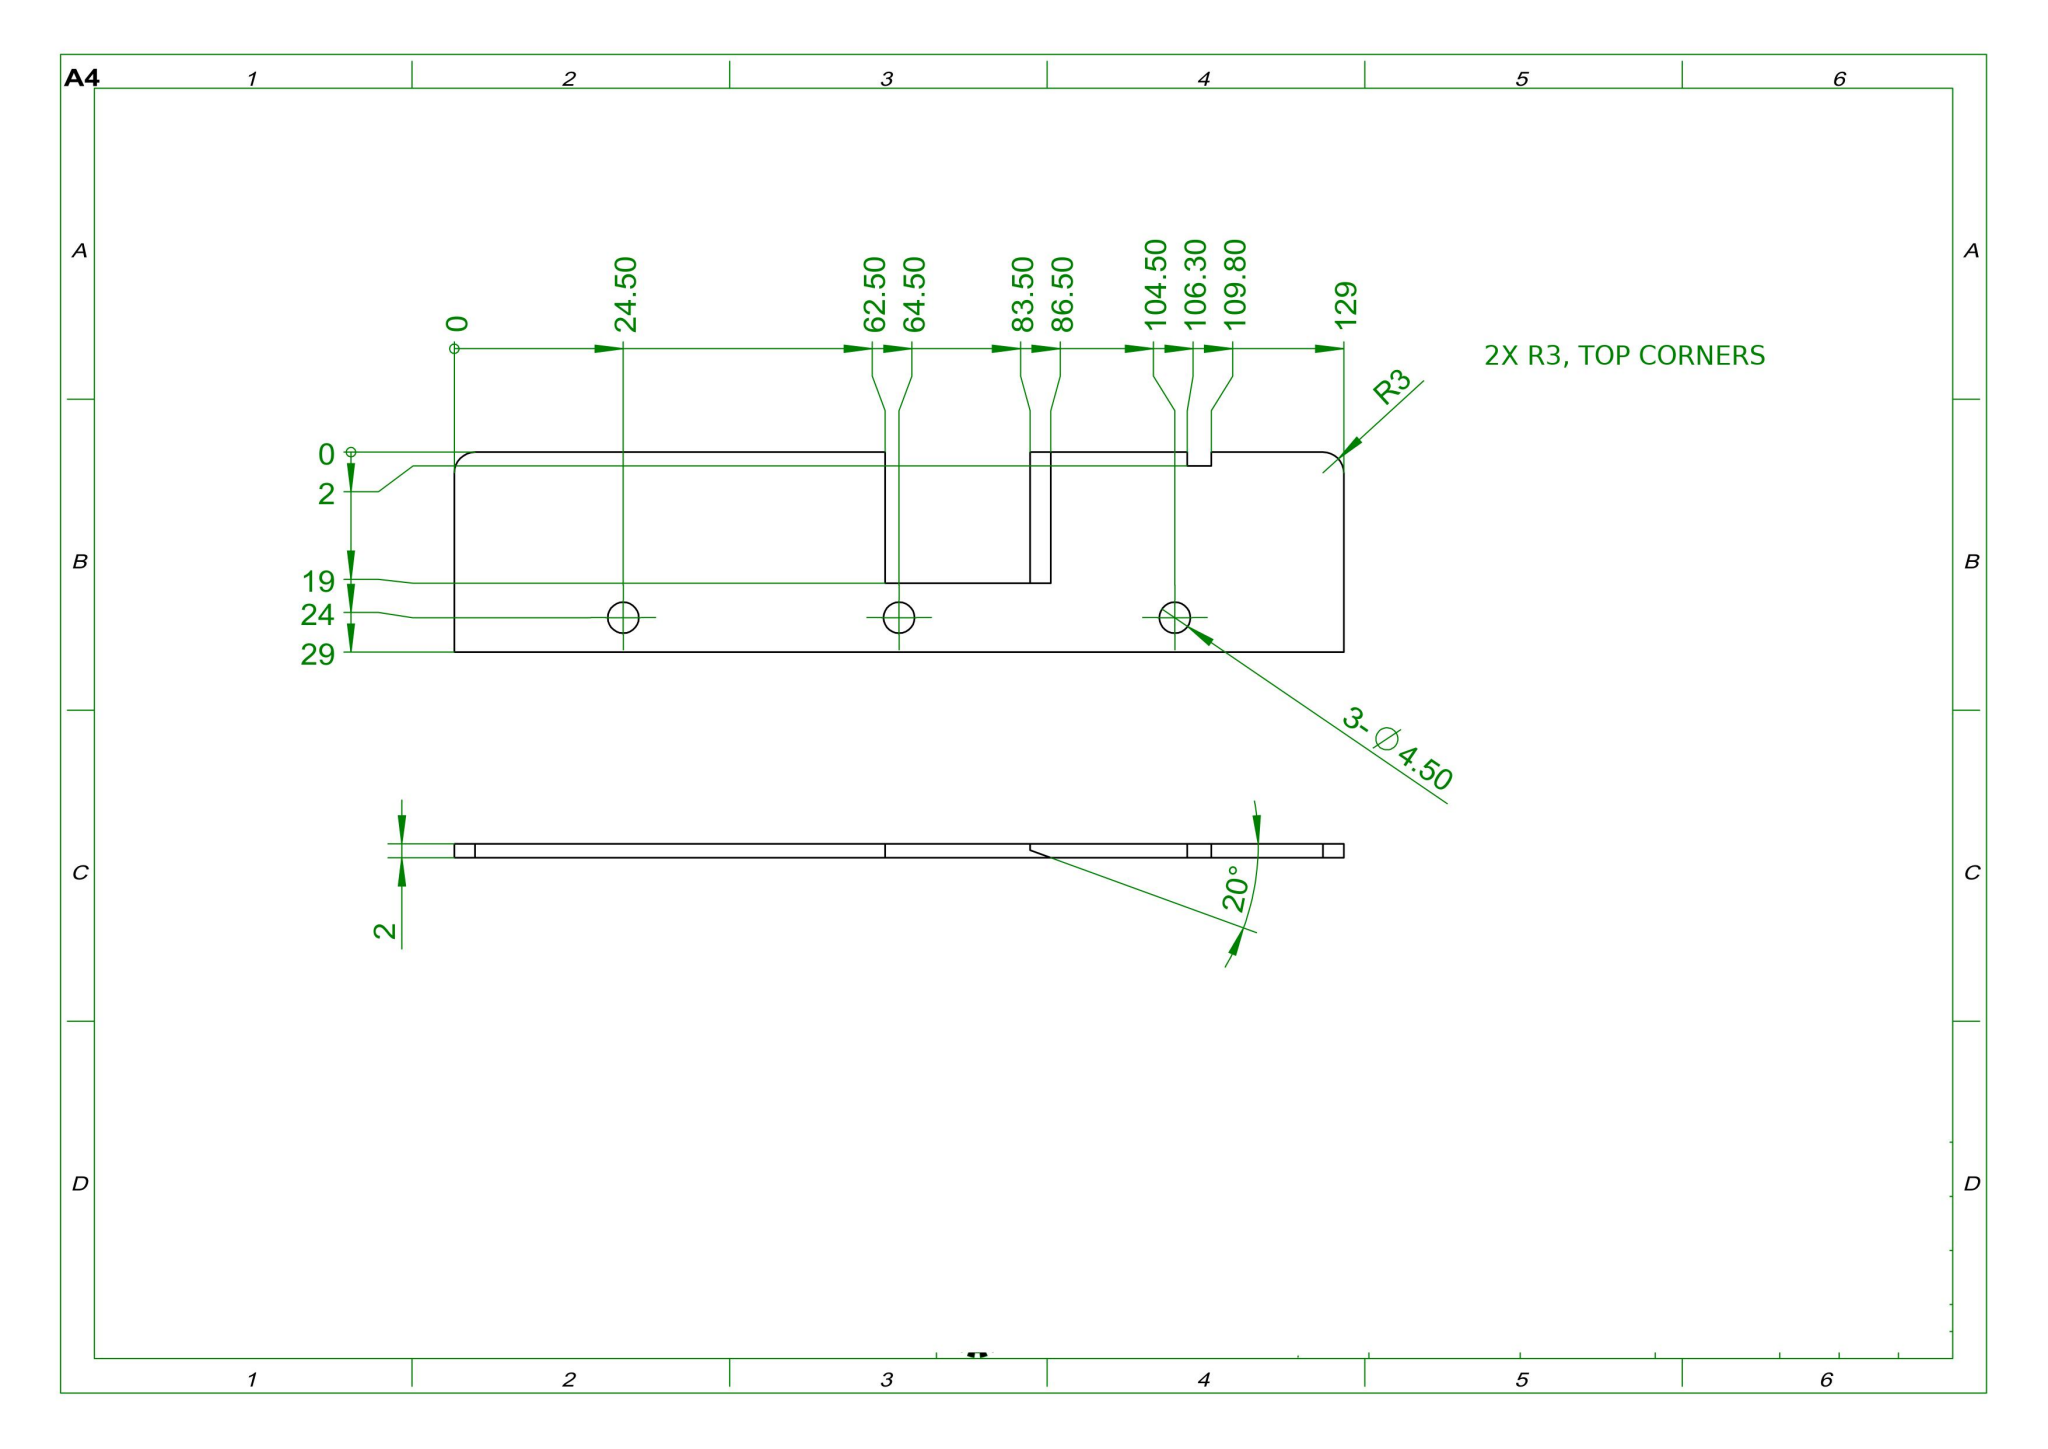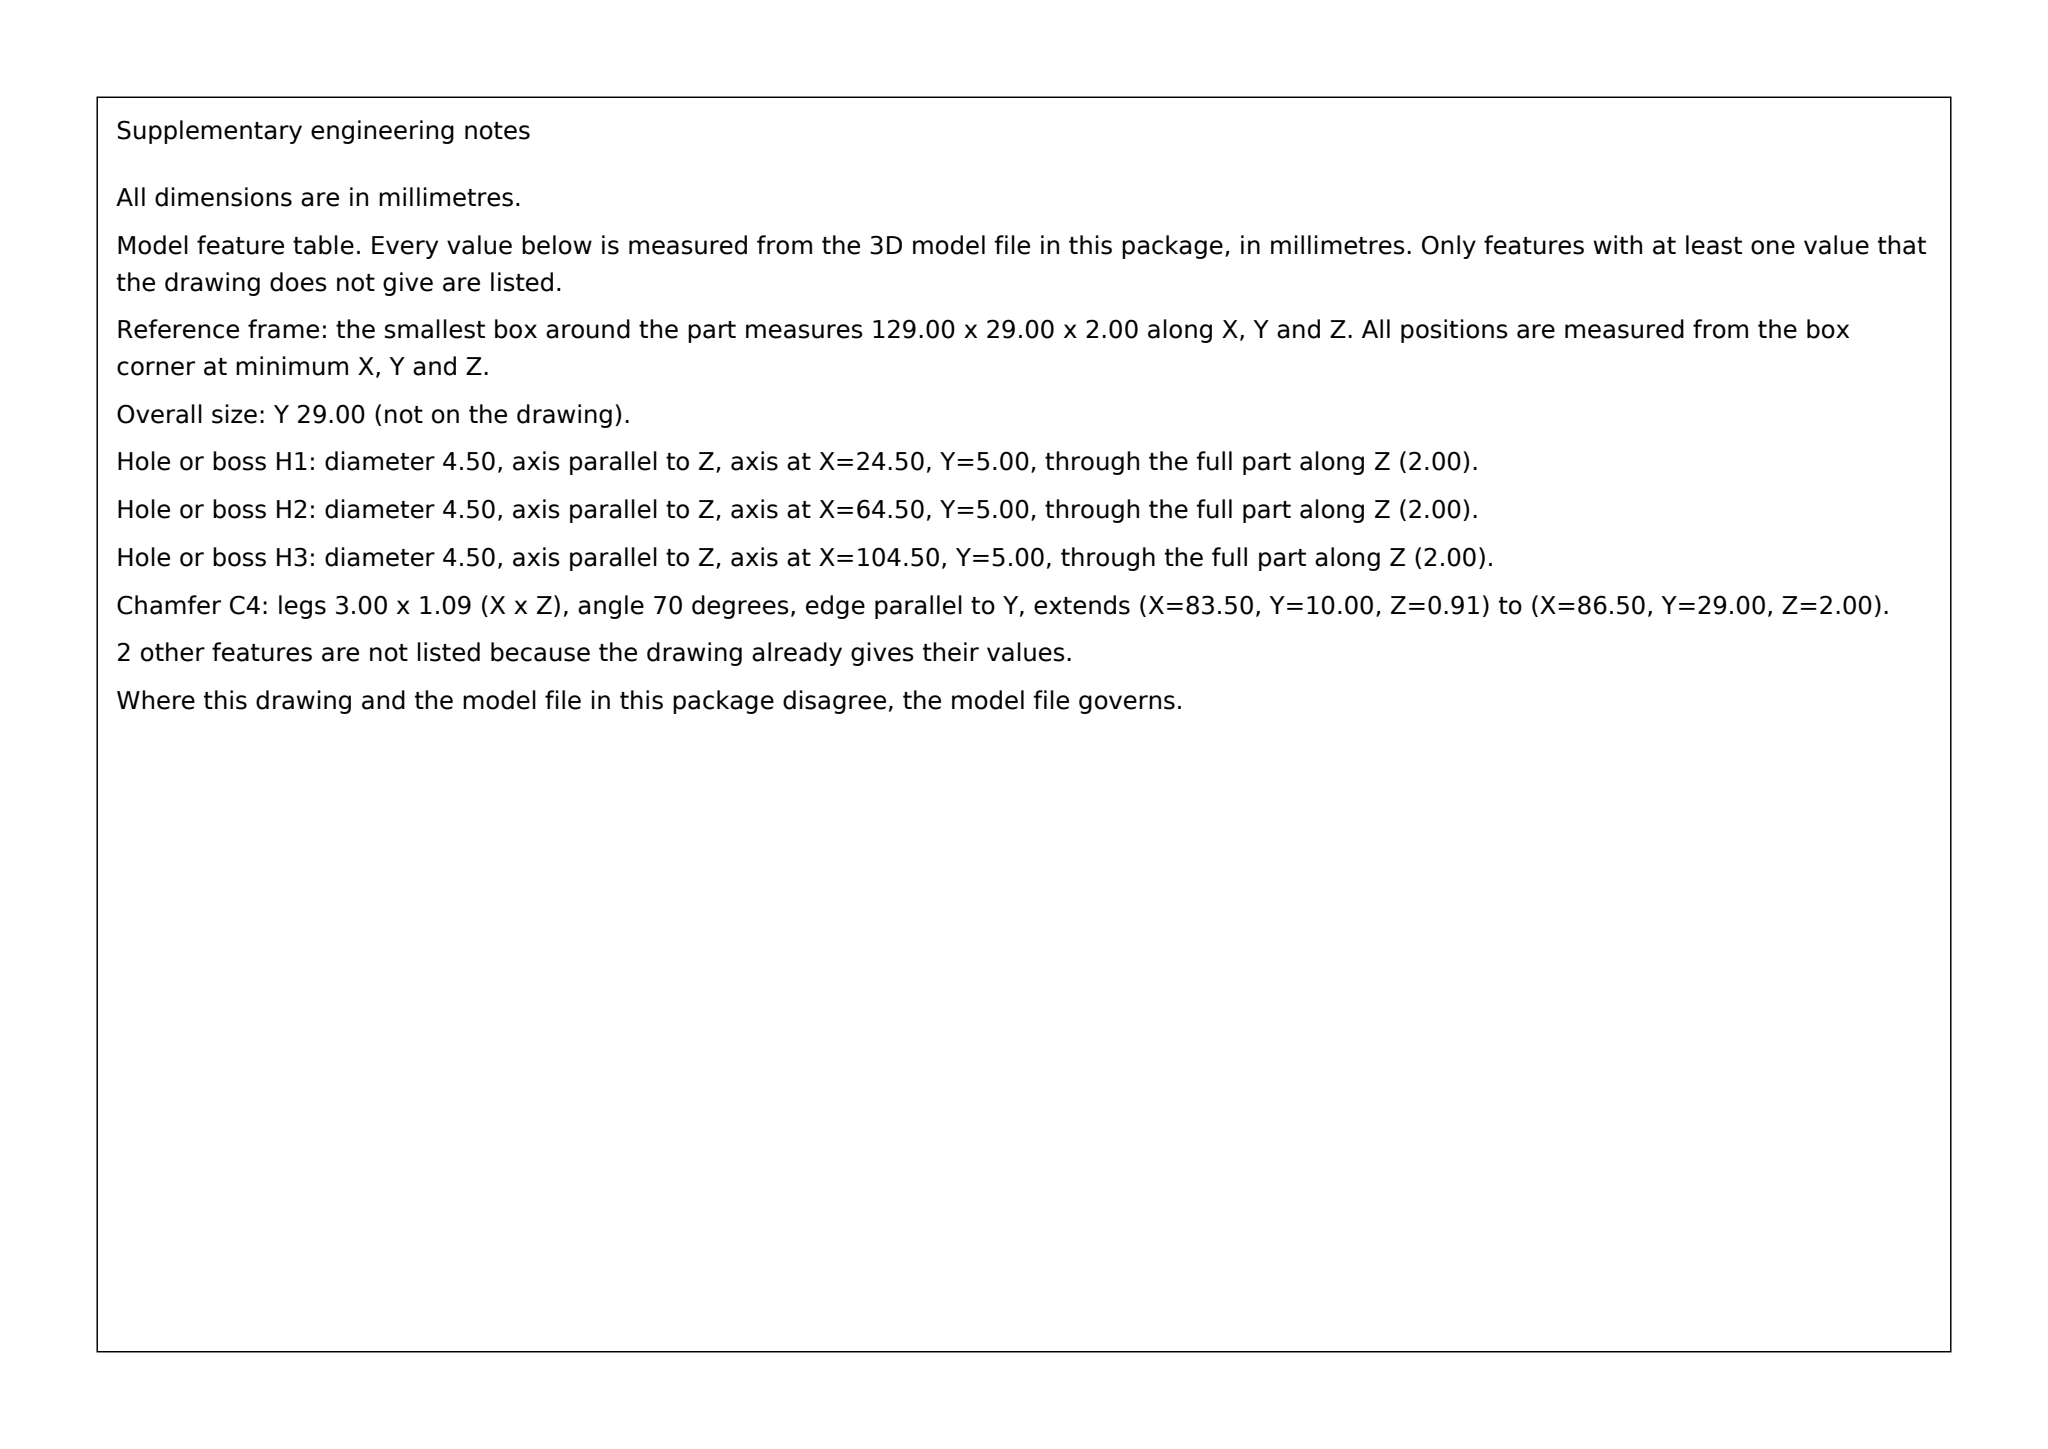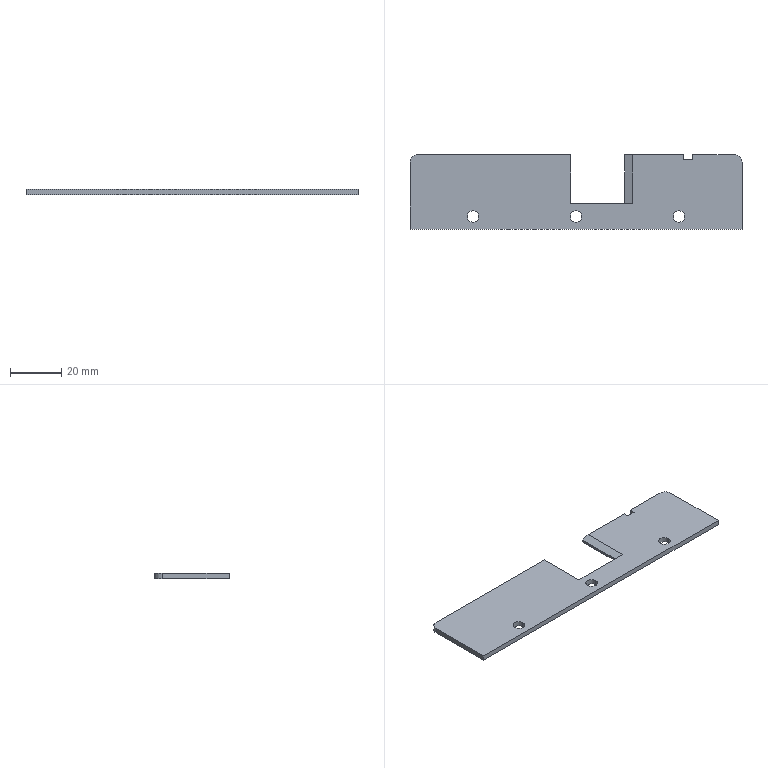Part | SolidWorks | mm | 1 solid | 23 faces | box 129 x 29 x 2 mm | volume 6536 mm3 | plane 15 | cylinder 8 | commonest cylinder face diameters 4.5 x6 6 x2
build123d program:
from build123d import *

# Parameters (mm, degrees)
SKETCH1_W           = 129
SKETCH1_H           = 29
BOSS_EXTRUDE1_DEPTH = 2
FILLET1_R           = 3
SKETCH2_W           = 21
SKETCH2_H           = 19
CUT_EXTRUDE1_DEPTH  = 2
CHAMFER1_SIZE       = 3
CHAMFER1_SIZE2      = 1.092
SKETCH3_R           = 2.25
CUT_EXTRUDE2_DEPTH  = 10
SKETCH4_W           = 3.5
SKETCH4_H           = 2
CUT_EXTRUDE3_DEPTH  = 2


with BuildPart() as part:
    # Sketch1 → Boss-Extrude1 (new body)
    with BuildSketch(Plane.XY):
        Rectangle(SKETCH1_W, SKETCH1_H)
    extrude(amount=BOSS_EXTRUDE1_DEPTH)

    # Fillet1
    fillet1_edges = [part.edges().sort_by_distance(p)[0] for p in [
        (-64.5, 14.5, 1),
        (64.5, 14.5, 1),
    ]]
    fillet(fillet1_edges, radius=FILLET1_R)

    # Sketch2 → Cut-Extrude1 (cut)
    with BuildSketch(Plane(origin=(0, 0, 0), x_dir=(-1, 0, 0), z_dir=(0, 0, -1))):
        with Locations((-8.5, 5)):
            Rectangle(SKETCH2_W, SKETCH2_H)
    extrude(amount=-CUT_EXTRUDE1_DEPTH, mode=Mode.SUBTRACT)

    # Chamfer1
    chamfer1_edges = [part.edges().sort_by_distance(p)[0] for p in [
        (19, 5, 2),
    ]]
    chamfer1_side = [part.faces().sort_by_distance(p)[0] for p in [
        (63.178, -1.5, 2),
    ]]
    chamfer(chamfer1_edges, length=CHAMFER1_SIZE, length2=CHAMFER1_SIZE2, reference=chamfer1_side[0])

    # Sketch3 → Cut-Extrude2 (cut)
    with BuildSketch(Plane(origin=(0, 0, 0), x_dir=(-1, 0, 0), z_dir=(0, 0, -1))):
        with Locations((0, -9.5)):
            Circle(SKETCH3_R)
        with Locations((-40, -9.5)):
            Circle(SKETCH3_R)
        with Locations((40, -9.5)):
            Circle(SKETCH3_R)
    extrude(amount=-CUT_EXTRUDE2_DEPTH, mode=Mode.SUBTRACT)

    # Sketch4 → Cut-Extrude3 (cut)
    with BuildSketch(Plane(origin=(0, 14.5, 0), x_dir=(1, 0, 0), z_dir=(0, 1, 0))):
        with Locations((43.55, -1)):
            Rectangle(SKETCH4_W, SKETCH4_H)
    extrude(amount=-CUT_EXTRUDE3_DEPTH, mode=Mode.SUBTRACT)


solid = part.part
STEP:
#1=CARTESIAN_POINT('',(-37.75,-9.5,2.));
#2=VERTEX_POINT('',#1);
#3=CARTESIAN_POINT('',(-42.25,-9.5,2.));
#4=VERTEX_POINT('',#3);
#5=CARTESIAN_POINT('',(-40.,-9.5,2.));
#6=DIRECTION('',(0.,0.,-1.));
#7=DIRECTION('',(-1.,0.,0.));
#8=AXIS2_PLACEMENT_3D('',#5,#6,#7);
#9=CIRCLE('',#8,2.25);
#10=EDGE_CURVE('',#2,#4,#9,.T.);
#11=ORIENTED_EDGE('',*,*,#10,.F.);
#12=CARTESIAN_POINT('',(-37.75,-9.5,0.));
#13=VERTEX_POINT('',#12);
#14=CARTESIAN_POINT('',(-37.75,-9.5,10.));
#15=DIRECTION('',(0.,0.,-1.));
#16=VECTOR('',#15,1000.);
#17=LINE('',#14,#16);
#18=EDGE_CURVE('',#2,#13,#17,.T.);
#19=ORIENTED_EDGE('',*,*,#18,.T.);
#20=CARTESIAN_POINT('',(-42.25,-9.5,0.));
#21=VERTEX_POINT('',#20);
#22=CARTESIAN_POINT('',(-40.,-9.5,0.));
#23=DIRECTION('',(0.,0.,-1.));
#24=DIRECTION('',(1.,0.,0.));
#25=AXIS2_PLACEMENT_3D('',#22,#23,#24);
#26=CIRCLE('',#25,2.25);
#27=EDGE_CURVE('',#13,#21,#26,.T.);
#28=ORIENTED_EDGE('',*,*,#27,.T.);
#29=CARTESIAN_POINT('',(-42.25,-9.5,10.));
#30=DIRECTION('',(0.,0.,-1.));
#31=VECTOR('',#30,1000.);
#32=LINE('',#29,#31);
#33=EDGE_CURVE('',#4,#21,#32,.T.);
#34=ORIENTED_EDGE('',*,*,#33,.F.);
#35=EDGE_LOOP('',(#11,#19,#28,#34));
#36=FACE_OUTER_BOUND('',#35,.T.);
#37=CARTESIAN_POINT('',(-40.,-9.5,10.));
#38=DIRECTION('',(0.,0.,-1.));
#39=DIRECTION('',(-1.,0.,0.));
#40=AXIS2_PLACEMENT_3D('',#37,#38,#39);
#41=CYLINDRICAL_SURFACE('',#40,2.25);
#42=ADVANCED_FACE('',(#36),#41,.F.);
#43=CARTESIAN_POINT('',(42.25,-9.5,2.));
#44=VERTEX_POINT('',#43);
#45=CARTESIAN_POINT('',(37.75,-9.5,2.));
#46=VERTEX_POINT('',#45);
#47=CARTESIAN_POINT('',(40.,-9.5,2.));
#48=DIRECTION('',(0.,0.,-1.));
#49=DIRECTION('',(-1.,0.,0.));
#50=AXIS2_PLACEMENT_3D('',#47,#48,#49);
#51=CIRCLE('',#50,2.25);
#52=EDGE_CURVE('',#44,#46,#51,.T.);
#53=ORIENTED_EDGE('',*,*,#52,.F.);
#54=CARTESIAN_POINT('',(42.25,-9.5,0.));
#55=VERTEX_POINT('',#54);
#56=CARTESIAN_POINT('',(42.25,-9.5,10.));
#57=DIRECTION('',(0.,0.,-1.));
#58=VECTOR('',#57,1000.);
#59=LINE('',#56,#58);
#60=EDGE_CURVE('',#44,#55,#59,.T.);
#61=ORIENTED_EDGE('',*,*,#60,.T.);
#62=CARTESIAN_POINT('',(37.75,-9.5,0.));
#63=VERTEX_POINT('',#62);
#64=CARTESIAN_POINT('',(40.,-9.5,0.));
#65=DIRECTION('',(0.,0.,-1.));
#66=DIRECTION('',(-1.,0.,0.));
#67=AXIS2_PLACEMENT_3D('',#64,#65,#66);
#68=CIRCLE('',#67,2.25);
#69=EDGE_CURVE('',#55,#63,#68,.T.);
#70=ORIENTED_EDGE('',*,*,#69,.T.);
#71=CARTESIAN_POINT('',(37.75,-9.5,10.));
#72=DIRECTION('',(0.,0.,-1.));
#73=VECTOR('',#72,1000.);
#74=LINE('',#71,#73);
#75=EDGE_CURVE('',#46,#63,#74,.T.);
#76=ORIENTED_EDGE('',*,*,#75,.F.);
#77=EDGE_LOOP('',(#53,#61,#70,#76));
#78=FACE_OUTER_BOUND('',#77,.T.);
#79=CARTESIAN_POINT('',(40.,-9.5,10.));
#80=DIRECTION('',(0.,0.,-1.));
#81=DIRECTION('',(-1.,0.,0.));
#82=AXIS2_PLACEMENT_3D('',#79,#80,#81);
#83=CYLINDRICAL_SURFACE('',#82,2.25);
#84=ADVANCED_FACE('',(#78),#83,.F.);
#85=CARTESIAN_POINT('',(2.25,-9.5,2.));
#86=VERTEX_POINT('',#85);
#87=CARTESIAN_POINT('',(-2.25,-9.5,2.));
#88=VERTEX_POINT('',#87);
#89=CARTESIAN_POINT('',(0.,-9.5,2.));
#90=DIRECTION('',(0.,0.,-1.));
#91=DIRECTION('',(-1.,0.,0.));
#92=AXIS2_PLACEMENT_3D('',#89,#90,#91);
#93=CIRCLE('',#92,2.25);
#94=EDGE_CURVE('',#86,#88,#93,.T.);
#95=ORIENTED_EDGE('',*,*,#94,.F.);
#96=CARTESIAN_POINT('',(2.25,-9.5,0.));
#97=VERTEX_POINT('',#96);
#98=CARTESIAN_POINT('',(2.25,-9.5,10.));
#99=DIRECTION('',(0.,0.,-1.));
#100=VECTOR('',#99,1000.);
#101=LINE('',#98,#100);
#102=EDGE_CURVE('',#86,#97,#101,.T.);
#103=ORIENTED_EDGE('',*,*,#102,.T.);
#104=CARTESIAN_POINT('',(-2.25,-9.5,0.));
#105=VERTEX_POINT('',#104);
#106=CARTESIAN_POINT('',(0.,-9.5,0.));
#107=DIRECTION('',(0.,0.,-1.));
#108=DIRECTION('',(-1.,0.,0.));
#109=AXIS2_PLACEMENT_3D('',#106,#107,#108);
#110=CIRCLE('',#109,2.25);
#111=EDGE_CURVE('',#97,#105,#110,.T.);
#112=ORIENTED_EDGE('',*,*,#111,.T.);
#113=CARTESIAN_POINT('',(-2.25,-9.5,10.));
#114=DIRECTION('',(0.,0.,-1.));
#115=VECTOR('',#114,1000.);
#116=LINE('',#113,#115);
#117=EDGE_CURVE('',#88,#105,#116,.T.);
#118=ORIENTED_EDGE('',*,*,#117,.F.);
#119=EDGE_LOOP('',(#95,#103,#112,#118));
#120=FACE_OUTER_BOUND('',#119,.T.);
#121=CARTESIAN_POINT('',(0.,-9.5,10.));
#122=DIRECTION('',(0.,0.,-1.));
#123=DIRECTION('',(-1.,0.,0.));
#124=AXIS2_PLACEMENT_3D('',#121,#122,#123);
#125=CYLINDRICAL_SURFACE('',#124,2.25);
#126=ADVANCED_FACE('',(#120),#125,.F.);
#127=CARTESIAN_POINT('',(41.8,14.5,2.));
#128=VERTEX_POINT('',#127);
#129=CARTESIAN_POINT('',(41.8,14.5,0.));
#130=VERTEX_POINT('',#129);
#131=CARTESIAN_POINT('',(41.8,14.5,2.));
#132=DIRECTION('',(0.,0.,-1.));
#133=VECTOR('',#132,1000.);
#134=LINE('',#131,#133);
#135=EDGE_CURVE('',#128,#130,#134,.T.);
#136=ORIENTED_EDGE('',*,*,#135,.T.);
#137=CARTESIAN_POINT('',(19.,14.5,0.));
#138=VERTEX_POINT('',#137);
#139=CARTESIAN_POINT('',(-64.5,14.5,0.));
#140=DIRECTION('',(-1.,0.,0.));
#141=VECTOR('',#140,1000.);
#142=LINE('',#139,#141);
#143=EDGE_CURVE('',#130,#138,#142,.T.);
#144=ORIENTED_EDGE('',*,*,#143,.T.);
#145=CARTESIAN_POINT('',(19.,14.5,0.9081));
#146=VERTEX_POINT('',#145);
#147=CARTESIAN_POINT('',(19.,14.5,2.));
#148=DIRECTION('',(0.,0.,-1.));
#149=VECTOR('',#148,1000.);
#150=LINE('',#147,#149);
#151=EDGE_CURVE('',#146,#138,#150,.T.);
#152=ORIENTED_EDGE('',*,*,#151,.F.);
#153=CARTESIAN_POINT('',(22.,14.5,2.));
#154=VERTEX_POINT('',#153);
#155=CARTESIAN_POINT('',(22.,14.5,2.));
#156=DIRECTION('',(0.9397,0.,0.342));
#157=VECTOR('',#156,1000.);
#158=LINE('',#155,#157);
#159=EDGE_CURVE('',#146,#154,#158,.T.);
#160=ORIENTED_EDGE('',*,*,#159,.T.);
#161=CARTESIAN_POINT('',(-64.5,14.5,2.));
#162=DIRECTION('',(-1.,0.,0.));
#163=VECTOR('',#162,1000.);
#164=LINE('',#161,#163);
#165=EDGE_CURVE('',#128,#154,#164,.T.);
#166=ORIENTED_EDGE('',*,*,#165,.F.);
#167=EDGE_LOOP('',(#136,#144,#152,#160,#166));
#168=FACE_OUTER_BOUND('',#167,.T.);
#169=CARTESIAN_POINT('',(-64.5,14.5,2.));
#170=DIRECTION('',(0.,-1.,0.));
#171=DIRECTION('',(0.,0.,-1.));
#172=AXIS2_PLACEMENT_3D('',#169,#170,#171);
#173=PLANE('',#172);
#174=ADVANCED_FACE('',(#168),#173,.F.);
#175=CARTESIAN_POINT('',(0.,-9.5,2.));
#176=DIRECTION('',(0.,0.,-1.));
#177=DIRECTION('',(-1.,0.,0.));
#178=AXIS2_PLACEMENT_3D('',#175,#176,#177);
#179=CIRCLE('',#178,2.25);
#180=EDGE_CURVE('',#88,#86,#179,.T.);
#181=ORIENTED_EDGE('',*,*,#180,.T.);
#182=ORIENTED_EDGE('',*,*,#94,.T.);
#183=EDGE_LOOP('',(#181,#182));
#184=FACE_BOUND('',#183,.T.);
#185=CARTESIAN_POINT('',(40.,-9.5,2.));
#186=DIRECTION('',(0.,0.,-1.));
#187=DIRECTION('',(-1.,0.,0.));
#188=AXIS2_PLACEMENT_3D('',#185,#186,#187);
#189=CIRCLE('',#188,2.25);
#190=EDGE_CURVE('',#46,#44,#189,.T.);
#191=ORIENTED_EDGE('',*,*,#190,.T.);
#192=ORIENTED_EDGE('',*,*,#52,.T.);
#193=EDGE_LOOP('',(#191,#192));
#194=FACE_BOUND('',#193,.T.);
#195=CARTESIAN_POINT('',(-40.,-9.5,2.));
#196=DIRECTION('',(0.,0.,-1.));
#197=DIRECTION('',(-1.,0.,0.));
#198=AXIS2_PLACEMENT_3D('',#195,#196,#197);
#199=CIRCLE('',#198,2.25);
#200=EDGE_CURVE('',#4,#2,#199,.T.);
#201=ORIENTED_EDGE('',*,*,#200,.T.);
#202=ORIENTED_EDGE('',*,*,#10,.T.);
#203=EDGE_LOOP('',(#201,#202));
#204=FACE_BOUND('',#203,.T.);
#205=CARTESIAN_POINT('',(41.8,12.5,2.));
#206=VERTEX_POINT('',#205);
#207=CARTESIAN_POINT('',(41.8,12.5,2.));
#208=DIRECTION('',(0.,1.,0.));
#209=VECTOR('',#208,1000.);
#210=LINE('',#207,#209);
#211=EDGE_CURVE('',#206,#128,#210,.T.);
#212=ORIENTED_EDGE('',*,*,#211,.T.);
#213=ORIENTED_EDGE('',*,*,#165,.T.);
#214=CARTESIAN_POINT('',(22.,-4.5,2.));
#215=VERTEX_POINT('',#214);
#216=CARTESIAN_POINT('',(22.,-0.,2.));
#217=DIRECTION('',(-0.,-1.,0.));
#218=VECTOR('',#217,1000.);
#219=LINE('',#216,#218);
#220=EDGE_CURVE('',#154,#215,#219,.T.);
#221=ORIENTED_EDGE('',*,*,#220,.T.);
#222=CARTESIAN_POINT('',(-2.,-4.5,2.));
#223=VERTEX_POINT('',#222);
#224=CARTESIAN_POINT('',(19.,-4.5,2.));
#225=DIRECTION('',(-1.,0.,0.));
#226=VECTOR('',#225,1000.);
#227=LINE('',#224,#226);
#228=EDGE_CURVE('',#215,#223,#227,.T.);
#229=ORIENTED_EDGE('',*,*,#228,.T.);
#230=CARTESIAN_POINT('',(-2.,14.5,2.));
#231=VERTEX_POINT('',#230);
#232=CARTESIAN_POINT('',(-2.,14.5,2.));
#233=DIRECTION('',(0.,1.,0.));
#234=VECTOR('',#233,1000.);
#235=LINE('',#232,#234);
#236=EDGE_CURVE('',#223,#231,#235,.T.);
#237=ORIENTED_EDGE('',*,*,#236,.T.);
#238=CARTESIAN_POINT('',(-61.5,14.5,2.));
#239=VERTEX_POINT('',#238);
#240=CARTESIAN_POINT('',(-64.5,14.5,2.));
#241=DIRECTION('',(-1.,0.,0.));
#242=VECTOR('',#241,1000.);
#243=LINE('',#240,#242);
#244=EDGE_CURVE('',#231,#239,#243,.T.);
#245=ORIENTED_EDGE('',*,*,#244,.T.);
#246=CARTESIAN_POINT('',(-64.5,11.5,2.));
#247=VERTEX_POINT('',#246);
#248=CARTESIAN_POINT('',(-61.5,11.5,2.));
#249=DIRECTION('',(0.,0.,1.));
#250=DIRECTION('',(-1.,0.,0.));
#251=AXIS2_PLACEMENT_3D('',#248,#249,#250);
#252=CIRCLE('',#251,3.);
#253=EDGE_CURVE('',#239,#247,#252,.T.);
#254=ORIENTED_EDGE('',*,*,#253,.T.);
#255=CARTESIAN_POINT('',(-64.5,-14.5,2.));
#256=VERTEX_POINT('',#255);
#257=CARTESIAN_POINT('',(-64.5,-14.5,2.));
#258=DIRECTION('',(0.,-1.,0.));
#259=VECTOR('',#258,1000.);
#260=LINE('',#257,#259);
#261=EDGE_CURVE('',#247,#256,#260,.T.);
#262=ORIENTED_EDGE('',*,*,#261,.T.);
#263=CARTESIAN_POINT('',(64.5,-14.5,2.));
#264=VERTEX_POINT('',#263);
#265=CARTESIAN_POINT('',(-64.5,-14.5,2.));
#266=DIRECTION('',(1.,0.,0.));
#267=VECTOR('',#266,1000.);
#268=LINE('',#265,#267);
#269=EDGE_CURVE('',#256,#264,#268,.T.);
#270=ORIENTED_EDGE('',*,*,#269,.T.);
#271=CARTESIAN_POINT('',(64.5,11.5,2.));
#272=VERTEX_POINT('',#271);
#273=CARTESIAN_POINT('',(64.5,-14.5,2.));
#274=DIRECTION('',(0.,1.,0.));
#275=VECTOR('',#274,1000.);
#276=LINE('',#273,#275);
#277=EDGE_CURVE('',#264,#272,#276,.T.);
#278=ORIENTED_EDGE('',*,*,#277,.T.);
#279=CARTESIAN_POINT('',(61.5,14.5,2.));
#280=VERTEX_POINT('',#279);
#281=CARTESIAN_POINT('',(61.5,11.5,2.));
#282=DIRECTION('',(0.,0.,1.));
#283=DIRECTION('',(-1.,0.,0.));
#284=AXIS2_PLACEMENT_3D('',#281,#282,#283);
#285=CIRCLE('',#284,3.);
#286=EDGE_CURVE('',#272,#280,#285,.T.);
#287=ORIENTED_EDGE('',*,*,#286,.T.);
#288=CARTESIAN_POINT('',(45.3,14.5,2.));
#289=VERTEX_POINT('',#288);
#290=CARTESIAN_POINT('',(-64.5,14.5,2.));
#291=DIRECTION('',(-1.,0.,0.));
#292=VECTOR('',#291,1000.);
#293=LINE('',#290,#292);
#294=EDGE_CURVE('',#280,#289,#293,.T.);
#295=ORIENTED_EDGE('',*,*,#294,.T.);
#296=CARTESIAN_POINT('',(45.3,12.5,2.));
#297=VERTEX_POINT('',#296);
#298=CARTESIAN_POINT('',(45.3,12.5,2.));
#299=DIRECTION('',(0.,1.,0.));
#300=VECTOR('',#299,1000.);
#301=LINE('',#298,#300);
#302=EDGE_CURVE('',#297,#289,#301,.T.);
#303=ORIENTED_EDGE('',*,*,#302,.F.);
#304=CARTESIAN_POINT('',(41.8,12.5,2.));
#305=DIRECTION('',(1.,0.,0.));
#306=VECTOR('',#305,1000.);
#307=LINE('',#304,#306);
#308=EDGE_CURVE('',#206,#297,#307,.T.);
#309=ORIENTED_EDGE('',*,*,#308,.F.);
#310=EDGE_LOOP('',(#212,#213,#221,#229,#237,#245,#254,#262,#270,#278,#287,#295,#303,#309));
#311=FACE_OUTER_BOUND('',#310,.T.);
#312=CARTESIAN_POINT('',(0.,0.,2.));
#313=DIRECTION('',(0.,0.,-1.));
#314=DIRECTION('',(-1.,0.,0.));
#315=AXIS2_PLACEMENT_3D('',#312,#313,#314);
#316=PLANE('',#315);
#317=ADVANCED_FACE('',(#184,#194,#204,#311),#316,.F.);
#318=CARTESIAN_POINT('',(0.,-9.5,0.));
#319=DIRECTION('',(0.,0.,-1.));
#320=DIRECTION('',(-1.,0.,0.));
#321=AXIS2_PLACEMENT_3D('',#318,#319,#320);
#322=CIRCLE('',#321,2.25);
#323=EDGE_CURVE('',#105,#97,#322,.T.);
#324=ORIENTED_EDGE('',*,*,#323,.F.);
#325=ORIENTED_EDGE('',*,*,#111,.F.);
#326=EDGE_LOOP('',(#324,#325));
#327=FACE_BOUND('',#326,.T.);
#328=CARTESIAN_POINT('',(40.,-9.5,0.));
#329=DIRECTION('',(0.,0.,-1.));
#330=DIRECTION('',(-1.,0.,0.));
#331=AXIS2_PLACEMENT_3D('',#328,#329,#330);
#332=CIRCLE('',#331,2.25);
#333=EDGE_CURVE('',#63,#55,#332,.T.);
#334=ORIENTED_EDGE('',*,*,#333,.F.);
#335=ORIENTED_EDGE('',*,*,#69,.F.);
#336=EDGE_LOOP('',(#334,#335));
#337=FACE_BOUND('',#336,.T.);
#338=CARTESIAN_POINT('',(-40.,-9.5,0.));
#339=DIRECTION('',(0.,0.,-1.));
#340=DIRECTION('',(1.,0.,0.));
#341=AXIS2_PLACEMENT_3D('',#338,#339,#340);
#342=CIRCLE('',#341,2.25);
#343=EDGE_CURVE('',#21,#13,#342,.T.);
#344=ORIENTED_EDGE('',*,*,#343,.F.);
#345=ORIENTED_EDGE('',*,*,#27,.F.);
#346=EDGE_LOOP('',(#344,#345));
#347=FACE_BOUND('',#346,.T.);
#348=ORIENTED_EDGE('',*,*,#143,.F.);
#349=CARTESIAN_POINT('',(41.8,12.5,0.));
#350=VERTEX_POINT('',#349);
#351=CARTESIAN_POINT('',(41.8,12.5,0.));
#352=DIRECTION('',(0.,1.,0.));
#353=VECTOR('',#352,1000.);
#354=LINE('',#351,#353);
#355=EDGE_CURVE('',#350,#130,#354,.T.);
#356=ORIENTED_EDGE('',*,*,#355,.F.);
#357=CARTESIAN_POINT('',(45.3,12.5,0.));
#358=VERTEX_POINT('',#357);
#359=CARTESIAN_POINT('',(41.8,12.5,0.));
#360=DIRECTION('',(1.,0.,0.));
#361=VECTOR('',#360,1000.);
#362=LINE('',#359,#361);
#363=EDGE_CURVE('',#350,#358,#362,.T.);
#364=ORIENTED_EDGE('',*,*,#363,.T.);
#365=CARTESIAN_POINT('',(45.3,14.5,0.));
#366=VERTEX_POINT('',#365);
#367=CARTESIAN_POINT('',(45.3,12.5,0.));
#368=DIRECTION('',(0.,1.,0.));
#369=VECTOR('',#368,1000.);
#370=LINE('',#367,#369);
#371=EDGE_CURVE('',#358,#366,#370,.T.);
#372=ORIENTED_EDGE('',*,*,#371,.T.);
#373=CARTESIAN_POINT('',(61.5,14.5,0.));
#374=VERTEX_POINT('',#373);
#375=CARTESIAN_POINT('',(-64.5,14.5,0.));
#376=DIRECTION('',(-1.,0.,0.));
#377=VECTOR('',#376,1000.);
#378=LINE('',#375,#377);
#379=EDGE_CURVE('',#374,#366,#378,.T.);
#380=ORIENTED_EDGE('',*,*,#379,.F.);
#381=CARTESIAN_POINT('',(64.5,11.5,0.));
#382=VERTEX_POINT('',#381);
#383=CARTESIAN_POINT('',(61.5,11.5,0.));
#384=DIRECTION('',(0.,0.,-1.));
#385=DIRECTION('',(-1.,0.,0.));
#386=AXIS2_PLACEMENT_3D('',#383,#384,#385);
#387=CIRCLE('',#386,3.);
#388=EDGE_CURVE('',#374,#382,#387,.T.);
#389=ORIENTED_EDGE('',*,*,#388,.T.);
#390=CARTESIAN_POINT('',(64.5,-14.5,0.));
#391=VERTEX_POINT('',#390);
#392=CARTESIAN_POINT('',(64.5,-14.5,0.));
#393=DIRECTION('',(0.,1.,0.));
#394=VECTOR('',#393,1000.);
#395=LINE('',#392,#394);
#396=EDGE_CURVE('',#391,#382,#395,.T.);
#397=ORIENTED_EDGE('',*,*,#396,.F.);
#398=CARTESIAN_POINT('',(-64.5,-14.5,0.));
#399=VERTEX_POINT('',#398);
#400=CARTESIAN_POINT('',(-64.5,-14.5,0.));
#401=DIRECTION('',(1.,0.,0.));
#402=VECTOR('',#401,1000.);
#403=LINE('',#400,#402);
#404=EDGE_CURVE('',#399,#391,#403,.T.);
#405=ORIENTED_EDGE('',*,*,#404,.F.);
#406=CARTESIAN_POINT('',(-64.5,11.5,0.));
#407=VERTEX_POINT('',#406);
#408=CARTESIAN_POINT('',(-64.5,-14.5,0.));
#409=DIRECTION('',(0.,-1.,0.));
#410=VECTOR('',#409,1000.);
#411=LINE('',#408,#410);
#412=EDGE_CURVE('',#407,#399,#411,.T.);
#413=ORIENTED_EDGE('',*,*,#412,.F.);
#414=CARTESIAN_POINT('',(-61.5,14.5,0.));
#415=VERTEX_POINT('',#414);
#416=CARTESIAN_POINT('',(-61.5,11.5,0.));
#417=DIRECTION('',(0.,0.,-1.));
#418=DIRECTION('',(-1.,0.,0.));
#419=AXIS2_PLACEMENT_3D('',#416,#417,#418);
#420=CIRCLE('',#419,3.);
#421=EDGE_CURVE('',#407,#415,#420,.T.);
#422=ORIENTED_EDGE('',*,*,#421,.T.);
#423=CARTESIAN_POINT('',(-2.,14.5,0.));
#424=VERTEX_POINT('',#423);
#425=CARTESIAN_POINT('',(-64.5,14.5,0.));
#426=DIRECTION('',(-1.,0.,0.));
#427=VECTOR('',#426,1000.);
#428=LINE('',#425,#427);
#429=EDGE_CURVE('',#424,#415,#428,.T.);
#430=ORIENTED_EDGE('',*,*,#429,.F.);
#431=CARTESIAN_POINT('',(-2.,-4.5,0.));
#432=VERTEX_POINT('',#431);
#433=CARTESIAN_POINT('',(-2.,14.5,0.));
#434=DIRECTION('',(0.,1.,0.));
#435=VECTOR('',#434,1000.);
#436=LINE('',#433,#435);
#437=EDGE_CURVE('',#432,#424,#436,.T.);
#438=ORIENTED_EDGE('',*,*,#437,.F.);
#439=CARTESIAN_POINT('',(19.,-4.5,0.));
#440=VERTEX_POINT('',#439);
#441=CARTESIAN_POINT('',(19.,-4.5,0.));
#442=DIRECTION('',(-1.,0.,0.));
#443=VECTOR('',#442,1000.);
#444=LINE('',#441,#443);
#445=EDGE_CURVE('',#440,#432,#444,.T.);
#446=ORIENTED_EDGE('',*,*,#445,.F.);
#447=CARTESIAN_POINT('',(19.,14.5,0.));
#448=DIRECTION('',(-0.,-1.,0.));
#449=VECTOR('',#448,1000.);
#450=LINE('',#447,#449);
#451=EDGE_CURVE('',#138,#440,#450,.T.);
#452=ORIENTED_EDGE('',*,*,#451,.F.);
#453=EDGE_LOOP('',(#348,#356,#364,#372,#380,#389,#397,#405,#413,#422,#430,#438,#446,#452));
#454=FACE_OUTER_BOUND('',#453,.T.);
#455=CARTESIAN_POINT('',(0.,0.,0.));
#456=DIRECTION('',(0.,0.,-1.));
#457=DIRECTION('',(-1.,0.,0.));
#458=AXIS2_PLACEMENT_3D('',#455,#456,#457);
#459=PLANE('',#458);
#460=ADVANCED_FACE('',(#327,#337,#347,#454),#459,.T.);
#461=ORIENTED_EDGE('',*,*,#379,.T.);
#462=CARTESIAN_POINT('',(45.3,14.5,2.));
#463=DIRECTION('',(0.,0.,-1.));
#464=VECTOR('',#463,1000.);
#465=LINE('',#462,#464);
#466=EDGE_CURVE('',#289,#366,#465,.T.);
#467=ORIENTED_EDGE('',*,*,#466,.F.);
#468=ORIENTED_EDGE('',*,*,#294,.F.);
#469=CARTESIAN_POINT('',(61.5,14.5,2.));
#470=DIRECTION('',(0.,0.,-1.));
#471=VECTOR('',#470,1000.);
#472=LINE('',#469,#471);
#473=EDGE_CURVE('',#280,#374,#472,.T.);
#474=ORIENTED_EDGE('',*,*,#473,.T.);
#475=EDGE_LOOP('',(#461,#467,#468,#474));
#476=FACE_OUTER_BOUND('',#475,.T.);
#477=CARTESIAN_POINT('',(-64.5,14.5,2.));
#478=DIRECTION('',(0.,-1.,0.));
#479=DIRECTION('',(0.,0.,-1.));
#480=AXIS2_PLACEMENT_3D('',#477,#478,#479);
#481=PLANE('',#480);
#482=ADVANCED_FACE('',(#476),#481,.F.);
#483=ORIENTED_EDGE('',*,*,#396,.T.);
#484=CARTESIAN_POINT('',(64.5,11.5,2.));
#485=DIRECTION('',(0.,0.,1.));
#486=VECTOR('',#485,1000.);
#487=LINE('',#484,#486);
#488=EDGE_CURVE('',#382,#272,#487,.T.);
#489=ORIENTED_EDGE('',*,*,#488,.T.);
#490=ORIENTED_EDGE('',*,*,#277,.F.);
#491=CARTESIAN_POINT('',(64.5,-14.5,2.));
#492=DIRECTION('',(0.,0.,-1.));
#493=VECTOR('',#492,1000.);
#494=LINE('',#491,#493);
#495=EDGE_CURVE('',#264,#391,#494,.T.);
#496=ORIENTED_EDGE('',*,*,#495,.T.);
#497=EDGE_LOOP('',(#483,#489,#490,#496));
#498=FACE_OUTER_BOUND('',#497,.T.);
#499=CARTESIAN_POINT('',(64.5,-14.5,2.));
#500=DIRECTION('',(-1.,0.,0.));
#501=DIRECTION('',(0.,0.,1.));
#502=AXIS2_PLACEMENT_3D('',#499,#500,#501);
#503=PLANE('',#502);
#504=ADVANCED_FACE('',(#498),#503,.F.);
#505=ORIENTED_EDGE('',*,*,#244,.F.);
#506=CARTESIAN_POINT('',(-2.,14.5,2.));
#507=DIRECTION('',(0.,0.,-1.));
#508=VECTOR('',#507,1000.);
#509=LINE('',#506,#508);
#510=EDGE_CURVE('',#231,#424,#509,.T.);
#511=ORIENTED_EDGE('',*,*,#510,.T.);
#512=ORIENTED_EDGE('',*,*,#429,.T.);
#513=CARTESIAN_POINT('',(-61.5,14.5,2.));
#514=DIRECTION('',(0.,0.,1.));
#515=VECTOR('',#514,1000.);
#516=LINE('',#513,#515);
#517=EDGE_CURVE('',#415,#239,#516,.T.);
#518=ORIENTED_EDGE('',*,*,#517,.T.);
#519=EDGE_LOOP('',(#505,#511,#512,#518));
#520=FACE_OUTER_BOUND('',#519,.T.);
#521=CARTESIAN_POINT('',(-64.5,14.5,2.));
#522=DIRECTION('',(0.,-1.,0.));
#523=DIRECTION('',(0.,0.,-1.));
#524=AXIS2_PLACEMENT_3D('',#521,#522,#523);
#525=PLANE('',#524);
#526=ADVANCED_FACE('',(#520),#525,.F.);
#527=ORIENTED_EDGE('',*,*,#261,.F.);
#528=CARTESIAN_POINT('',(-64.5,11.5,2.));
#529=DIRECTION('',(0.,0.,-1.));
#530=VECTOR('',#529,1000.);
#531=LINE('',#528,#530);
#532=EDGE_CURVE('',#247,#407,#531,.T.);
#533=ORIENTED_EDGE('',*,*,#532,.T.);
#534=ORIENTED_EDGE('',*,*,#412,.T.);
#535=CARTESIAN_POINT('',(-64.5,-14.5,2.));
#536=DIRECTION('',(0.,0.,-1.));
#537=VECTOR('',#536,1000.);
#538=LINE('',#535,#537);
#539=EDGE_CURVE('',#256,#399,#538,.T.);
#540=ORIENTED_EDGE('',*,*,#539,.F.);
#541=EDGE_LOOP('',(#527,#533,#534,#540));
#542=FACE_OUTER_BOUND('',#541,.T.);
#543=CARTESIAN_POINT('',(-64.5,-14.5,2.));
#544=DIRECTION('',(1.,0.,0.));
#545=DIRECTION('',(0.,0.,-1.));
#546=AXIS2_PLACEMENT_3D('',#543,#544,#545);
#547=PLANE('',#546);
#548=ADVANCED_FACE('',(#542),#547,.F.);
#549=ORIENTED_EDGE('',*,*,#404,.T.);
#550=ORIENTED_EDGE('',*,*,#495,.F.);
#551=ORIENTED_EDGE('',*,*,#269,.F.);
#552=ORIENTED_EDGE('',*,*,#539,.T.);
#553=EDGE_LOOP('',(#549,#550,#551,#552));
#554=FACE_OUTER_BOUND('',#553,.T.);
#555=CARTESIAN_POINT('',(-64.5,-14.5,2.));
#556=DIRECTION('',(0.,1.,0.));
#557=DIRECTION('',(0.,0.,1.));
#558=AXIS2_PLACEMENT_3D('',#555,#556,#557);
#559=PLANE('',#558);
#560=ADVANCED_FACE('',(#554),#559,.F.);
#561=ORIENTED_EDGE('',*,*,#286,.F.);
#562=ORIENTED_EDGE('',*,*,#488,.F.);
#563=ORIENTED_EDGE('',*,*,#388,.F.);
#564=ORIENTED_EDGE('',*,*,#473,.F.);
#565=EDGE_LOOP('',(#561,#562,#563,#564));
#566=FACE_OUTER_BOUND('',#565,.T.);
#567=CARTESIAN_POINT('',(61.5,11.5,2.));
#568=DIRECTION('',(0.,0.,-1.));
#569=DIRECTION('',(-1.,0.,0.));
#570=AXIS2_PLACEMENT_3D('',#567,#568,#569);
#571=CYLINDRICAL_SURFACE('',#570,3.);
#572=ADVANCED_FACE('',(#566),#571,.T.);
#573=ORIENTED_EDGE('',*,*,#253,.F.);
#574=ORIENTED_EDGE('',*,*,#517,.F.);
#575=ORIENTED_EDGE('',*,*,#421,.F.);
#576=ORIENTED_EDGE('',*,*,#532,.F.);
#577=EDGE_LOOP('',(#573,#574,#575,#576));
#578=FACE_OUTER_BOUND('',#577,.T.);
#579=CARTESIAN_POINT('',(-61.5,11.5,2.));
#580=DIRECTION('',(0.,0.,-1.));
#581=DIRECTION('',(-1.,0.,0.));
#582=AXIS2_PLACEMENT_3D('',#579,#580,#581);
#583=CYLINDRICAL_SURFACE('',#582,3.);
#584=ADVANCED_FACE('',(#578),#583,.T.);
#585=CARTESIAN_POINT('',(19.,-4.5,0.9081));
#586=VERTEX_POINT('',#585);
#587=CARTESIAN_POINT('',(19.,-4.5,2.));
#588=DIRECTION('',(0.,0.,-1.));
#589=VECTOR('',#588,1000.);
#590=LINE('',#587,#589);
#591=EDGE_CURVE('',#586,#440,#590,.T.);
#592=ORIENTED_EDGE('',*,*,#591,.F.);
#593=CARTESIAN_POINT('',(19.,14.5,0.9081));
#594=DIRECTION('',(0.,1.,0.));
#595=VECTOR('',#594,1000.);
#596=LINE('',#593,#595);
#597=EDGE_CURVE('',#586,#146,#596,.T.);
#598=ORIENTED_EDGE('',*,*,#597,.T.);
#599=ORIENTED_EDGE('',*,*,#151,.T.);
#600=ORIENTED_EDGE('',*,*,#451,.T.);
#601=EDGE_LOOP('',(#592,#598,#599,#600));
#602=FACE_OUTER_BOUND('',#601,.T.);
#603=CARTESIAN_POINT('',(19.,14.5,2.));
#604=DIRECTION('',(1.,-0.,0.));
#605=DIRECTION('',(0.,1.,0.));
#606=AXIS2_PLACEMENT_3D('',#603,#604,#605);
#607=PLANE('',#606);
#608=ADVANCED_FACE('',(#602),#607,.F.);
#609=ORIENTED_EDGE('',*,*,#437,.T.);
#610=ORIENTED_EDGE('',*,*,#510,.F.);
#611=ORIENTED_EDGE('',*,*,#236,.F.);
#612=CARTESIAN_POINT('',(-2.,-4.5,2.));
#613=DIRECTION('',(0.,0.,-1.));
#614=VECTOR('',#613,1000.);
#615=LINE('',#612,#614);
#616=EDGE_CURVE('',#223,#432,#615,.T.);
#617=ORIENTED_EDGE('',*,*,#616,.T.);
#618=EDGE_LOOP('',(#609,#610,#611,#617));
#619=FACE_OUTER_BOUND('',#618,.T.);
#620=CARTESIAN_POINT('',(-2.,14.5,2.));
#621=DIRECTION('',(-1.,0.,0.));
#622=DIRECTION('',(-0.,-1.,0.));
#623=AXIS2_PLACEMENT_3D('',#620,#621,#622);
#624=PLANE('',#623);
#625=ADVANCED_FACE('',(#619),#624,.F.);
#626=ORIENTED_EDGE('',*,*,#445,.T.);
#627=ORIENTED_EDGE('',*,*,#616,.F.);
#628=ORIENTED_EDGE('',*,*,#228,.F.);
#629=CARTESIAN_POINT('',(19.351,-4.5,1.036));
#630=DIRECTION('',(-0.9397,0.,-0.342));
#631=VECTOR('',#630,1000.);
#632=LINE('',#629,#631);
#633=EDGE_CURVE('',#215,#586,#632,.T.);
#634=ORIENTED_EDGE('',*,*,#633,.T.);
#635=ORIENTED_EDGE('',*,*,#591,.T.);
#636=EDGE_LOOP('',(#626,#627,#628,#634,#635));
#637=FACE_OUTER_BOUND('',#636,.T.);
#638=CARTESIAN_POINT('',(19.,-4.5,2.));
#639=DIRECTION('',(-0.,-1.,0.));
#640=DIRECTION('',(1.,-0.,0.));
#641=AXIS2_PLACEMENT_3D('',#638,#639,#640);
#642=PLANE('',#641);
#643=ADVANCED_FACE('',(#637),#642,.F.);
#644=ORIENTED_EDGE('',*,*,#159,.F.);
#645=ORIENTED_EDGE('',*,*,#597,.F.);
#646=ORIENTED_EDGE('',*,*,#633,.F.);
#647=ORIENTED_EDGE('',*,*,#220,.F.);
#648=EDGE_LOOP('',(#644,#645,#646,#647));
#649=FACE_OUTER_BOUND('',#648,.T.);
#650=CARTESIAN_POINT('',(22.,-0.,2.));
#651=DIRECTION('',(0.342,-0.,-0.9397));
#652=DIRECTION('',(-0.,-1.,0.));
#653=AXIS2_PLACEMENT_3D('',#650,#651,#652);
#654=PLANE('',#653);
#655=ADVANCED_FACE('',(#649),#654,.F.);
#656=ORIENTED_EDGE('',*,*,#102,.F.);
#657=ORIENTED_EDGE('',*,*,#180,.F.);
#658=ORIENTED_EDGE('',*,*,#117,.T.);
#659=ORIENTED_EDGE('',*,*,#323,.T.);
#660=EDGE_LOOP('',(#656,#657,#658,#659));
#661=FACE_OUTER_BOUND('',#660,.T.);
#662=CARTESIAN_POINT('',(0.,-9.5,10.));
#663=DIRECTION('',(0.,0.,-1.));
#664=DIRECTION('',(-1.,0.,0.));
#665=AXIS2_PLACEMENT_3D('',#662,#663,#664);
#666=CYLINDRICAL_SURFACE('',#665,2.25);
#667=ADVANCED_FACE('',(#661),#666,.F.);
#668=ORIENTED_EDGE('',*,*,#60,.F.);
#669=ORIENTED_EDGE('',*,*,#190,.F.);
#670=ORIENTED_EDGE('',*,*,#75,.T.);
#671=ORIENTED_EDGE('',*,*,#333,.T.);
#672=EDGE_LOOP('',(#668,#669,#670,#671));
#673=FACE_OUTER_BOUND('',#672,.T.);
#674=CARTESIAN_POINT('',(40.,-9.5,10.));
#675=DIRECTION('',(0.,0.,-1.));
#676=DIRECTION('',(-1.,0.,0.));
#677=AXIS2_PLACEMENT_3D('',#674,#675,#676);
#678=CYLINDRICAL_SURFACE('',#677,2.25);
#679=ADVANCED_FACE('',(#673),#678,.F.);
#680=ORIENTED_EDGE('',*,*,#18,.F.);
#681=ORIENTED_EDGE('',*,*,#200,.F.);
#682=ORIENTED_EDGE('',*,*,#33,.T.);
#683=ORIENTED_EDGE('',*,*,#343,.T.);
#684=EDGE_LOOP('',(#680,#681,#682,#683));
#685=FACE_OUTER_BOUND('',#684,.T.);
#686=CARTESIAN_POINT('',(-40.,-9.5,10.));
#687=DIRECTION('',(0.,0.,-1.));
#688=DIRECTION('',(-1.,0.,0.));
#689=AXIS2_PLACEMENT_3D('',#686,#687,#688);
#690=CYLINDRICAL_SURFACE('',#689,2.25);
#691=ADVANCED_FACE('',(#685),#690,.F.);
#692=ORIENTED_EDGE('',*,*,#135,.F.);
#693=ORIENTED_EDGE('',*,*,#211,.F.);
#694=CARTESIAN_POINT('',(41.8,12.5,2.));
#695=DIRECTION('',(0.,0.,-1.));
#696=VECTOR('',#695,1000.);
#697=LINE('',#694,#696);
#698=EDGE_CURVE('',#206,#350,#697,.T.);
#699=ORIENTED_EDGE('',*,*,#698,.T.);
#700=ORIENTED_EDGE('',*,*,#355,.T.);
#701=EDGE_LOOP('',(#692,#693,#699,#700));
#702=FACE_OUTER_BOUND('',#701,.T.);
#703=CARTESIAN_POINT('',(41.8,12.5,2.));
#704=DIRECTION('',(1.,0.,0.));
#705=DIRECTION('',(0.,0.,-1.));
#706=AXIS2_PLACEMENT_3D('',#703,#704,#705);
#707=PLANE('',#706);
#708=ADVANCED_FACE('',(#702),#707,.T.);
#709=ORIENTED_EDGE('',*,*,#466,.T.);
#710=ORIENTED_EDGE('',*,*,#371,.F.);
#711=CARTESIAN_POINT('',(45.3,12.5,2.));
#712=DIRECTION('',(0.,0.,-1.));
#713=VECTOR('',#712,1000.);
#714=LINE('',#711,#713);
#715=EDGE_CURVE('',#297,#358,#714,.T.);
#716=ORIENTED_EDGE('',*,*,#715,.F.);
#717=ORIENTED_EDGE('',*,*,#302,.T.);
#718=EDGE_LOOP('',(#709,#710,#716,#717));
#719=FACE_OUTER_BOUND('',#718,.T.);
#720=CARTESIAN_POINT('',(45.3,12.5,2.));
#721=DIRECTION('',(1.,0.,0.));
#722=DIRECTION('',(0.,0.,-1.));
#723=AXIS2_PLACEMENT_3D('',#720,#721,#722);
#724=PLANE('',#723);
#725=ADVANCED_FACE('',(#719),#724,.F.);
#726=ORIENTED_EDGE('',*,*,#308,.T.);
#727=ORIENTED_EDGE('',*,*,#715,.T.);
#728=ORIENTED_EDGE('',*,*,#363,.F.);
#729=ORIENTED_EDGE('',*,*,#698,.F.);
#730=EDGE_LOOP('',(#726,#727,#728,#729));
#731=FACE_OUTER_BOUND('',#730,.T.);
#732=CARTESIAN_POINT('',(0.,12.5,0.));
#733=DIRECTION('',(0.,1.,0.));
#734=DIRECTION('',(0.,0.,1.));
#735=AXIS2_PLACEMENT_3D('',#732,#733,#734);
#736=PLANE('',#735);
#737=ADVANCED_FACE('',(#731),#736,.T.);
#738=CLOSED_SHELL('',(#42,#84,#126,#174,#317,#460,#482,#504,#526,#548,#560,#572,#584,#608,#625,#643,#655,#667,#679,#691,#708,#725,#737));
#739=MANIFOLD_SOLID_BREP('',#738);
#740=CARTESIAN_POINT('',(0.,0.,0.));
#741=DIRECTION('',(0.,0.,1.));
#742=DIRECTION('',(1.,0.,0.));
#743=AXIS2_PLACEMENT_3D('',#740,#741,#742);
#744=(LENGTH_UNIT()NAMED_UNIT(*)SI_UNIT(.MILLI.,.METRE.));
#745=UNCERTAINTY_MEASURE_WITH_UNIT(LENGTH_MEASURE(0.00001),#744,'','');
#746=(NAMED_UNIT(*)PLANE_ANGLE_UNIT()SI_UNIT($,.RADIAN.));
#747=(NAMED_UNIT(*)SI_UNIT($,.STERADIAN.)SOLID_ANGLE_UNIT());
#748=(GEOMETRIC_REPRESENTATION_CONTEXT(3)GLOBAL_UNCERTAINTY_ASSIGNED_CONTEXT((#745))GLOBAL_UNIT_ASSIGNED_CONTEXT((#744,#746,#747))REPRESENTATION_CONTEXT('',''));
#749=ADVANCED_BREP_SHAPE_REPRESENTATION('',(#739,#743),#748);